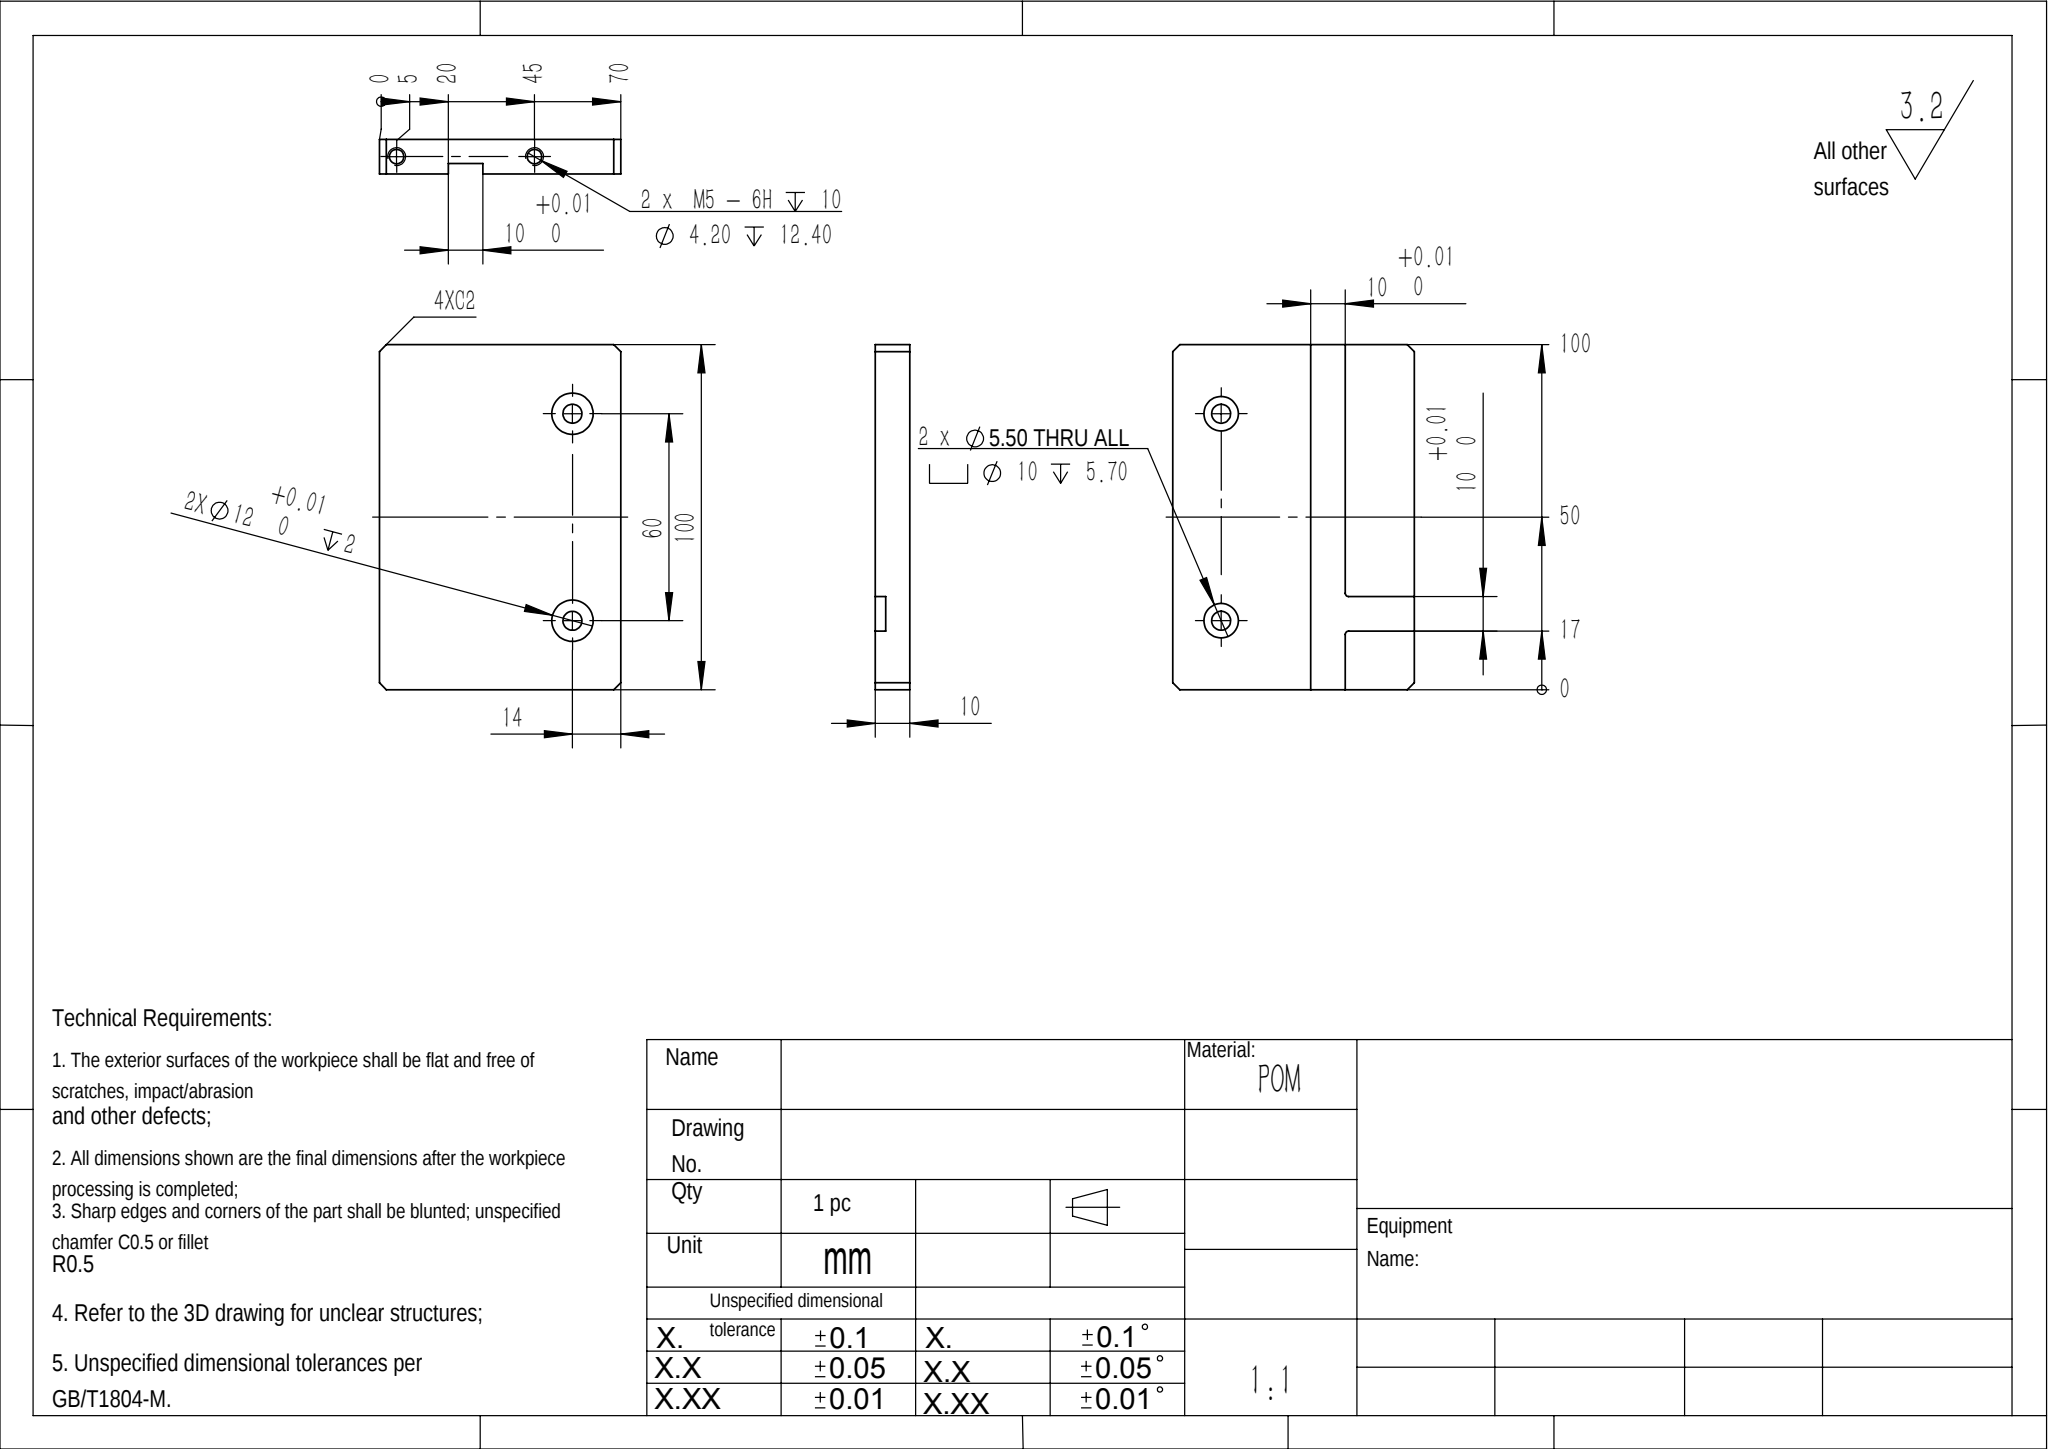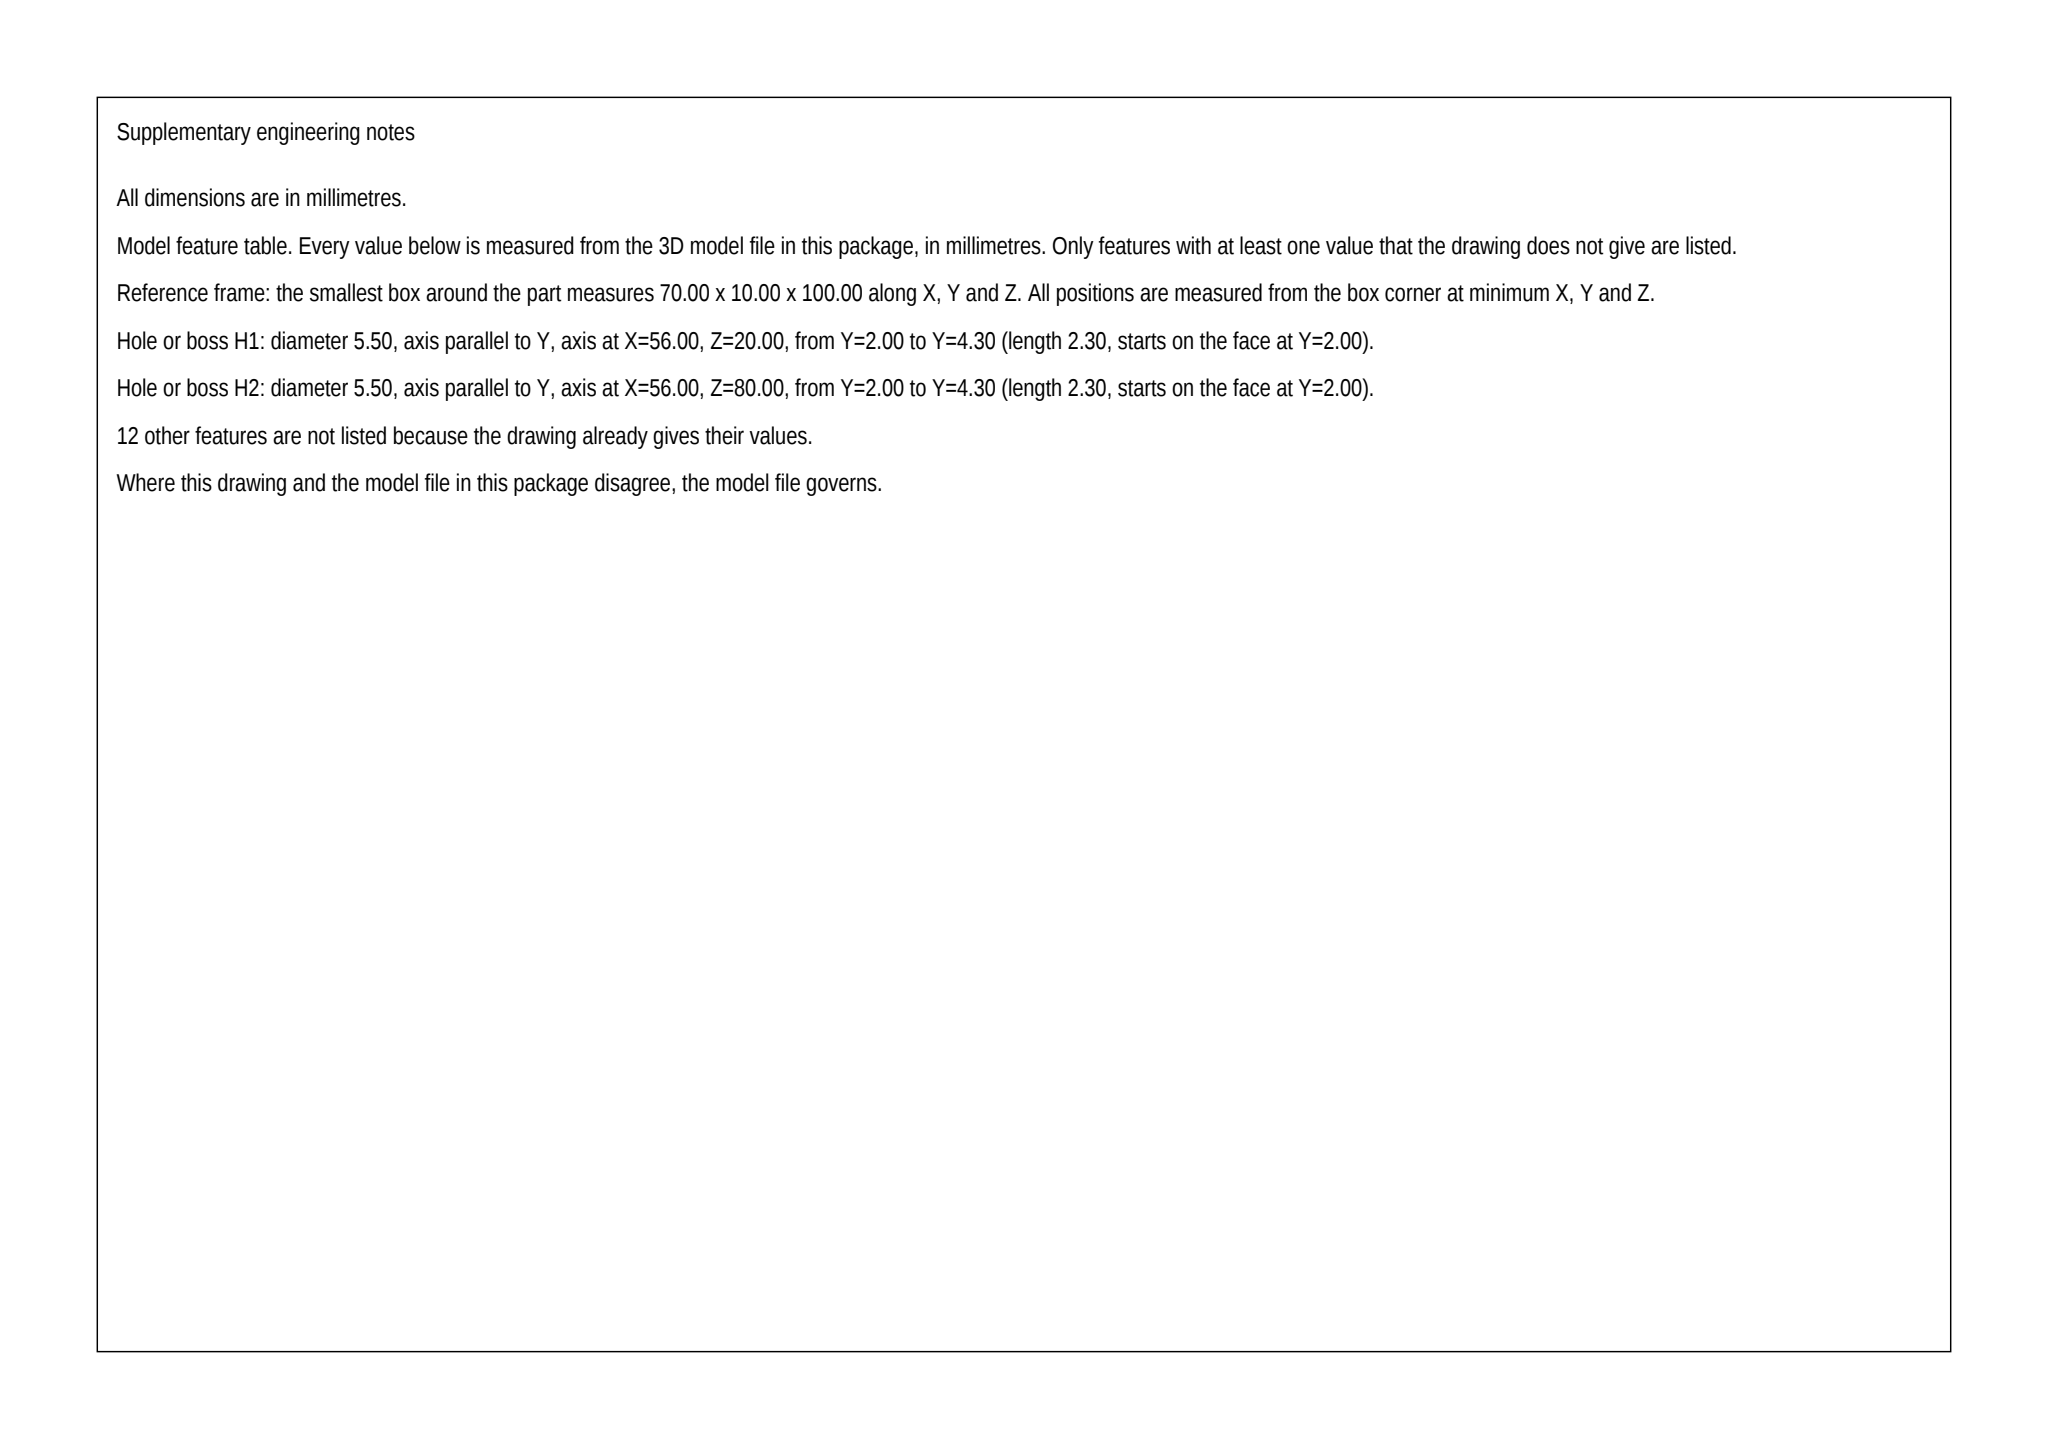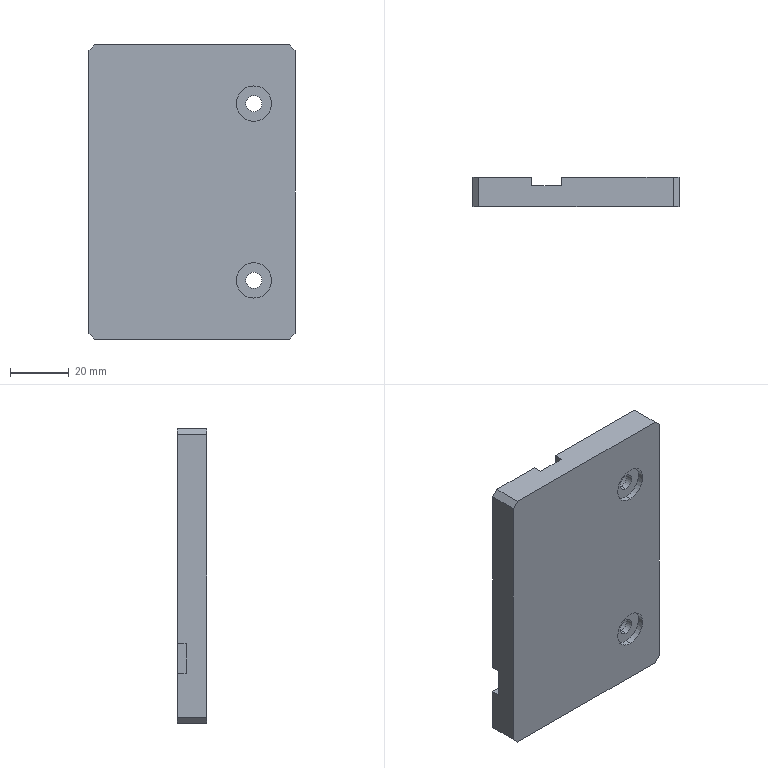Part | SolidWorks | mm | material POM | 1 solid | 44 faces | box 70 x 10 x 100 mm | volume 64506 mm3 | plane 22 | cylinder 18 | cone 4 | commonest cylinder face diameters 12 x4 10 x4 4.2 x4 5.5 x4 2 x2
Drawing notes:
BACK FACE RECESS 3 DEEP, 7 THK REMAINING | from the solid: y planes at 7.0 and 10.0; bbox y=10 -> 3 mm cut to y=7 face
2X R1 FILLET AT SLOT CORNERS (Z17 & Z27, 19 FROM LH EDGE) | from the solid: Convex arcs dia 2.0 (R1), axis y, at (x19,z16) and (x19,z28), y7-10, 90 deg; adjacent planes z=17 and z=27 (x 0-19) and x=20 walls
build123d program:
from build123d import *

# Parameters (mm, degrees)
SKETCH1_W                                         = 70
SKETCH1_H                                         = 100
BOSS_EXTRUDE1_DEPTH                               = 10
CUT_EXTRUDE3_DEPTH                                = 3
M5_TAPPED_HOLE1_D                                 = 4.2
M5_TAPPED_HOLE1_DEPTH                             = 12.4
M5_TAPPED_HOLE1_TIP                               = 1.262
HOLE_SIZE_ACCORDING_TO_HEXAGON_SOCKET_D           = 5.5
HOLE_SIZE_ACCORDING_TO_HEXAGON_SOCKET_CBORE_D     = 10
HOLE_SIZE_ACCORDING_TO_HEXAGON_SOCKET_CBORE_DEPTH = 5.7
SKETCH23_R                                        = 6
CUT_EXTRUDE5_DEPTH                                = 2
CHAMFER1_SIZE                                     = 2
FILLET1_R                                         = 1


with BuildPart() as part:
    # Sketch1 → Boss-Extrude1 (new body)
    with BuildSketch(Plane(origin=(0, 0, 0), x_dir=(1, 0, 0), z_dir=(0, 1, 0))):
        Rectangle(SKETCH1_W, SKETCH1_H)
    extrude(amount=BOSS_EXTRUDE1_DEPTH)

    # Sketch6 → Cut-Extrude3 (cut)
    with BuildSketch(Plane(origin=(0, 10, 0), x_dir=(1, 0, 0), z_dir=(0, 1, 0))):
        Polygon((-15, -50), (-5, -50), (-5, 50), (-15, 50), (-15, 33), (-35, 33), (-35, 23), (-15, 23), align=None)
    extrude(amount=-CUT_EXTRUDE3_DEPTH, mode=Mode.SUBTRACT)

    # M5 Tapped Hole1
    with Locations(Plane(origin=(-30, 5, -50), x_dir=(-1, 0, 0), z_dir=(0, 0, -1))):
        with Locations((0, 0), (-40, 0)):
            Hole(M5_TAPPED_HOLE1_D / 2, depth=M5_TAPPED_HOLE1_DEPTH)
            with Locations((0, 0, -(M5_TAPPED_HOLE1_DEPTH + M5_TAPPED_HOLE1_TIP / 2))):  # 118° drill point
                Cone(0, M5_TAPPED_HOLE1_D / 2, M5_TAPPED_HOLE1_TIP, mode=Mode.SUBTRACT)

    # Hole Size _ according to_ Hexagon Socket (through all)
    with Locations(Plane(origin=(21, 10, 30), x_dir=(0, 0, 1), z_dir=(0, 1, 0))):
        with Locations((0, 0), (-60, 0)):
            CounterBoreHole(HOLE_SIZE_ACCORDING_TO_HEXAGON_SOCKET_D / 2, HOLE_SIZE_ACCORDING_TO_HEXAGON_SOCKET_CBORE_D / 2, HOLE_SIZE_ACCORDING_TO_HEXAGON_SOCKET_CBORE_DEPTH)

    # Sketch23 → Cut-Extrude5 (cut)
    with BuildSketch(Plane.XZ):
        with Locations(Location((21, 30, 0), (0, 0, 270))):
            Circle(SKETCH23_R)
        with Locations(Location((21, -30, 0), (0, 0, 270))):
            Circle(SKETCH23_R)
    extrude(amount=-CUT_EXTRUDE5_DEPTH, mode=Mode.SUBTRACT)

    # Chamfer1
    chamfer1_edges = [part.edges().sort_by_distance(p)[0] for p in [
        (35, 5, 50),
        (-35, 5, 50),
        (-35, 5, -50),
        (35, 5, -50),
    ]]
    chamfer(chamfer1_edges, length=CHAMFER1_SIZE)

    # Fillet1
    fillet1_edges = [part.edges().sort_by_distance(p)[0] for p in [
        (-15, 8.5, -23),
        (-15, 8.5, -33),
    ]]
    fillet(fillet1_edges, radius=FILLET1_R)


solid = part.part